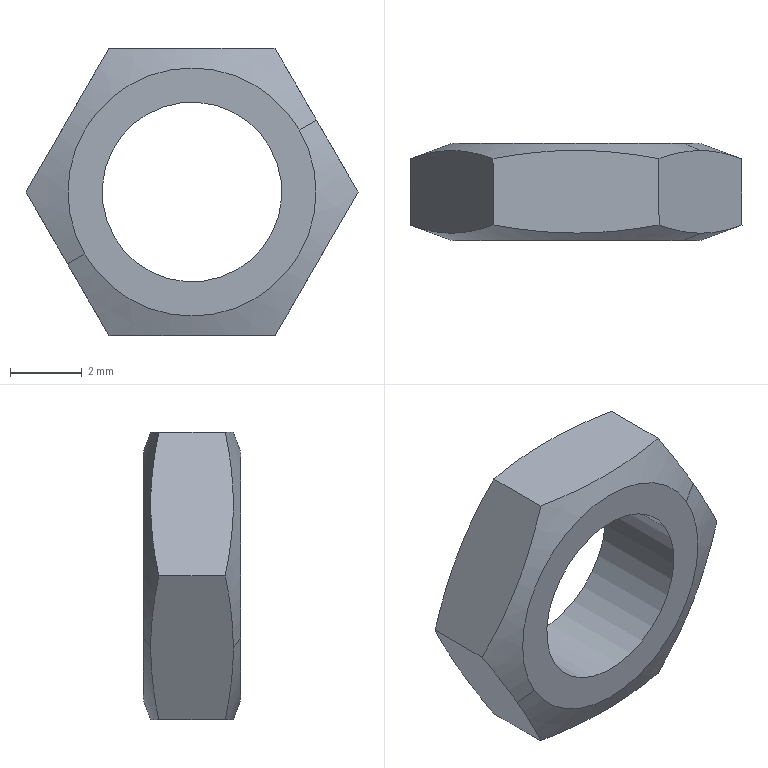Component | SolidWorks | 18M5StainlessSteelNut-1 | 1 solid | 14 faces | box 9.24 x 2.7 x 8 mm | volume 91 mm3 | plane 8 | cone 4 | cylinder 2 | commonest cylinder face diameters 5 x2 | material SUS304
STEP:
#1=CARTESIAN_POINT('',(-0.6207,1.188,3.061));
#2=VERTEX_POINT('',#1);
#3=CARTESIAN_POINT('',(-0.4502,1.188,3.159));
#4=VERTEX_POINT('',#3);
#5=CARTESIAN_POINT('',(-0.5354,1.188,3.11));
#6=DIRECTION('',(0.,-1.,0.));
#7=DIRECTION('',(0.866,0.,0.5));
#8=AXIS2_PLACEMENT_3D('',#5,#6,#7);
#9=CIRCLE('',#8,0.09843);
#10=EDGE_CURVE('',#2,#4,#9,.T.);
#11=ORIENTED_EDGE('',*,*,#10,.F.);
#12=CARTESIAN_POINT('',(-0.6207,1.082,3.061));
#13=VERTEX_POINT('',#12);
#14=CARTESIAN_POINT('',(-0.6207,1.188,3.061));
#15=DIRECTION('',(0.,-1.,0.));
#16=VECTOR('',#15,39.37);
#17=LINE('',#14,#16);
#18=EDGE_CURVE('',#2,#13,#17,.T.);
#19=ORIENTED_EDGE('',*,*,#18,.T.);
#20=CARTESIAN_POINT('',(-0.4502,1.082,3.159));
#21=VERTEX_POINT('',#20);
#22=CARTESIAN_POINT('',(-0.5354,1.082,3.11));
#23=DIRECTION('',(0.,-1.,0.));
#24=DIRECTION('',(0.866,0.,0.5));
#25=AXIS2_PLACEMENT_3D('',#22,#23,#24);
#26=CIRCLE('',#25,0.09843);
#27=EDGE_CURVE('',#13,#21,#26,.T.);
#28=ORIENTED_EDGE('',*,*,#27,.T.);
#29=CARTESIAN_POINT('',(-0.4502,1.188,3.159));
#30=DIRECTION('',(0.,-1.,0.));
#31=VECTOR('',#30,39.37);
#32=LINE('',#29,#31);
#33=EDGE_CURVE('',#4,#21,#32,.T.);
#34=ORIENTED_EDGE('',*,*,#33,.F.);
#35=EDGE_LOOP('',(#11,#19,#28,#34));
#36=FACE_OUTER_BOUND('',#35,.T.);
#37=CARTESIAN_POINT('',(-0.5354,1.188,3.11));
#38=DIRECTION('',(0.,-1.,0.));
#39=DIRECTION('',(0.866,0.,0.5));
#40=AXIS2_PLACEMENT_3D('',#37,#38,#39);
#41=CYLINDRICAL_SURFACE('',#40,0.09843);
#42=ADVANCED_FACE('',(#36),#41,.F.);
#43=CARTESIAN_POINT('',(-0.4178,1.082,3.178));
#44=VERTEX_POINT('',#43);
#45=CARTESIAN_POINT('',(-0.653,1.082,3.042));
#46=VERTEX_POINT('',#45);
#47=CARTESIAN_POINT('',(-0.5354,1.082,3.11));
#48=DIRECTION('',(0.,-1.,0.));
#49=DIRECTION('',(-0.866,0.,-0.5));
#50=AXIS2_PLACEMENT_3D('',#47,#48,#49);
#51=CIRCLE('',#50,0.1358);
#52=EDGE_CURVE('',#44,#46,#51,.T.);
#53=ORIENTED_EDGE('',*,*,#52,.F.);
#54=CARTESIAN_POINT('',(-0.399,1.089,3.189));
#55=VERTEX_POINT('',#54);
#56=CARTESIAN_POINT('',(-0.3777,1.098,3.201));
#57=DIRECTION('',(0.8138,0.342,0.4698));
#58=VECTOR('',#57,39.37);
#59=LINE('',#56,#58);
#60=EDGE_CURVE('',#44,#55,#59,.T.);
#61=ORIENTED_EDGE('',*,*,#60,.T.);
#62=CARTESIAN_POINT('',(-0.4445,1.098,3.268));
#63=VERTEX_POINT('',#62);
#64=CARTESIAN_POINT('',(-0.399,1.089,3.189));
#65=CARTESIAN_POINT('',(-0.4142,1.089,3.215));
#66=CARTESIAN_POINT('',(-0.4293,1.093,3.241));
#67=CARTESIAN_POINT('',(-0.4445,1.098,3.268));
#68=B_SPLINE_CURVE_WITH_KNOTS('',3,(#64,#65,#66,#67),.UNSPECIFIED.,.F.,.F.,(4,4),(0.002309,0.004619),.UNSPECIFIED.);
#69=EDGE_CURVE('',#55,#63,#68,.T.);
#70=ORIENTED_EDGE('',*,*,#69,.T.);
#71=CARTESIAN_POINT('',(-0.6263,1.098,3.268));
#72=VERTEX_POINT('',#71);
#73=CARTESIAN_POINT('',(-0.4445,1.098,3.268));
#74=CARTESIAN_POINT('',(-0.4748,1.093,3.268));
#75=CARTESIAN_POINT('',(-0.5354,1.086,3.268));
#76=CARTESIAN_POINT('',(-0.596,1.093,3.268));
#77=CARTESIAN_POINT('',(-0.6263,1.098,3.268));
#78=B_SPLINE_CURVE_WITH_KNOTS('',3,(#73,#74,#75,#76,#77),.UNSPECIFIED.,.F.,.F.,(4,1,4),(0.,0.002309,0.004619),.UNSPECIFIED.);
#79=EDGE_CURVE('',#63,#72,#78,.T.);
#80=ORIENTED_EDGE('',*,*,#79,.T.);
#81=CARTESIAN_POINT('',(-0.7173,1.098,3.11));
#82=VERTEX_POINT('',#81);
#83=CARTESIAN_POINT('',(-0.6263,1.098,3.268));
#84=CARTESIAN_POINT('',(-0.6415,1.093,3.241));
#85=CARTESIAN_POINT('',(-0.6718,1.086,3.189));
#86=CARTESIAN_POINT('',(-0.7021,1.093,3.136));
#87=CARTESIAN_POINT('',(-0.7173,1.098,3.11));
#88=B_SPLINE_CURVE_WITH_KNOTS('',3,(#83,#84,#85,#86,#87),.UNSPECIFIED.,.F.,.F.,(4,1,4),(0.,0.002309,0.004619),.UNSPECIFIED.);
#89=EDGE_CURVE('',#72,#82,#88,.T.);
#90=ORIENTED_EDGE('',*,*,#89,.T.);
#91=CARTESIAN_POINT('',(-0.6718,1.089,3.031));
#92=VERTEX_POINT('',#91);
#93=CARTESIAN_POINT('',(-0.7173,1.098,3.11));
#94=CARTESIAN_POINT('',(-0.7021,1.093,3.084));
#95=CARTESIAN_POINT('',(-0.687,1.089,3.058));
#96=CARTESIAN_POINT('',(-0.6718,1.089,3.031));
#97=B_SPLINE_CURVE_WITH_KNOTS('',3,(#93,#94,#95,#96),.UNSPECIFIED.,.F.,.F.,(4,4),(0.,0.002309),.UNSPECIFIED.);
#98=EDGE_CURVE('',#82,#92,#97,.T.);
#99=ORIENTED_EDGE('',*,*,#98,.T.);
#100=CARTESIAN_POINT('',(-0.6931,1.098,3.019));
#101=DIRECTION('',(-0.8138,0.342,-0.4698));
#102=VECTOR('',#101,39.37);
#103=LINE('',#100,#102);
#104=EDGE_CURVE('',#46,#92,#103,.T.);
#105=ORIENTED_EDGE('',*,*,#104,.F.);
#106=EDGE_LOOP('',(#53,#61,#70,#80,#90,#99,#105));
#107=FACE_OUTER_BOUND('',#106,.T.);
#108=CARTESIAN_POINT('',(-0.5354,1.098,3.11));
#109=DIRECTION('',(-0.,1.,-0.));
#110=DIRECTION('',(-0.866,0.,-0.5));
#111=AXIS2_PLACEMENT_3D('',#108,#109,#110);
#112=CONICAL_SURFACE('',#111,0.1821,1.222);
#113=ADVANCED_FACE('',(#107),#112,.T.);
#114=CARTESIAN_POINT('',(-0.4178,1.188,3.178));
#115=VERTEX_POINT('',#114);
#116=CARTESIAN_POINT('',(-0.653,1.188,3.042));
#117=VERTEX_POINT('',#116);
#118=CARTESIAN_POINT('',(-0.5354,1.188,3.11));
#119=DIRECTION('',(0.,-1.,0.));
#120=DIRECTION('',(0.866,0.,0.5));
#121=AXIS2_PLACEMENT_3D('',#118,#119,#120);
#122=CIRCLE('',#121,0.1358);
#123=EDGE_CURVE('',#115,#117,#122,.T.);
#124=ORIENTED_EDGE('',*,*,#123,.T.);
#125=CARTESIAN_POINT('',(-0.6718,1.18,3.031));
#126=VERTEX_POINT('',#125);
#127=CARTESIAN_POINT('',(-0.6931,1.171,3.019));
#128=DIRECTION('',(-0.8138,-0.342,-0.4698));
#129=VECTOR('',#128,39.37);
#130=LINE('',#127,#129);
#131=EDGE_CURVE('',#117,#126,#130,.T.);
#132=ORIENTED_EDGE('',*,*,#131,.T.);
#133=CARTESIAN_POINT('',(-0.7173,1.171,3.11));
#134=VERTEX_POINT('',#133);
#135=CARTESIAN_POINT('',(-0.6718,1.18,3.031));
#136=CARTESIAN_POINT('',(-0.687,1.18,3.058));
#137=CARTESIAN_POINT('',(-0.7021,1.177,3.084));
#138=CARTESIAN_POINT('',(-0.7173,1.171,3.11));
#139=B_SPLINE_CURVE_WITH_KNOTS('',3,(#135,#136,#137,#138),.UNSPECIFIED.,.F.,.F.,(4,4),(0.002309,0.004619),.UNSPECIFIED.);
#140=EDGE_CURVE('',#126,#134,#139,.T.);
#141=ORIENTED_EDGE('',*,*,#140,.T.);
#142=CARTESIAN_POINT('',(-0.6263,1.171,3.268));
#143=VERTEX_POINT('',#142);
#144=CARTESIAN_POINT('',(-0.7173,1.171,3.11));
#145=CARTESIAN_POINT('',(-0.7021,1.177,3.136));
#146=CARTESIAN_POINT('',(-0.6718,1.183,3.189));
#147=CARTESIAN_POINT('',(-0.6415,1.177,3.241));
#148=CARTESIAN_POINT('',(-0.6263,1.171,3.268));
#149=B_SPLINE_CURVE_WITH_KNOTS('',3,(#144,#145,#146,#147,#148),.UNSPECIFIED.,.F.,.F.,(4,1,4),(0.,0.002309,0.004619),.UNSPECIFIED.);
#150=EDGE_CURVE('',#134,#143,#149,.T.);
#151=ORIENTED_EDGE('',*,*,#150,.T.);
#152=CARTESIAN_POINT('',(-0.4445,1.171,3.268));
#153=VERTEX_POINT('',#152);
#154=CARTESIAN_POINT('',(-0.6263,1.171,3.268));
#155=CARTESIAN_POINT('',(-0.596,1.177,3.268));
#156=CARTESIAN_POINT('',(-0.5354,1.183,3.268));
#157=CARTESIAN_POINT('',(-0.4748,1.177,3.268));
#158=CARTESIAN_POINT('',(-0.4445,1.171,3.268));
#159=B_SPLINE_CURVE_WITH_KNOTS('',3,(#154,#155,#156,#157,#158),.UNSPECIFIED.,.F.,.F.,(4,1,4),(0.,0.002309,0.004619),.UNSPECIFIED.);
#160=EDGE_CURVE('',#143,#153,#159,.T.);
#161=ORIENTED_EDGE('',*,*,#160,.T.);
#162=CARTESIAN_POINT('',(-0.399,1.18,3.189));
#163=VERTEX_POINT('',#162);
#164=CARTESIAN_POINT('',(-0.4445,1.171,3.268));
#165=CARTESIAN_POINT('',(-0.4293,1.177,3.241));
#166=CARTESIAN_POINT('',(-0.4142,1.18,3.215));
#167=CARTESIAN_POINT('',(-0.399,1.18,3.189));
#168=B_SPLINE_CURVE_WITH_KNOTS('',3,(#164,#165,#166,#167),.UNSPECIFIED.,.F.,.F.,(4,4),(0.,0.002309),.UNSPECIFIED.);
#169=EDGE_CURVE('',#153,#163,#168,.T.);
#170=ORIENTED_EDGE('',*,*,#169,.T.);
#171=CARTESIAN_POINT('',(-0.3777,1.171,3.201));
#172=DIRECTION('',(0.8138,-0.342,0.4698));
#173=VECTOR('',#172,39.37);
#174=LINE('',#171,#173);
#175=EDGE_CURVE('',#115,#163,#174,.T.);
#176=ORIENTED_EDGE('',*,*,#175,.F.);
#177=EDGE_LOOP('',(#124,#132,#141,#151,#161,#170,#176));
#178=FACE_OUTER_BOUND('',#177,.T.);
#179=CARTESIAN_POINT('',(-0.5354,1.171,3.11));
#180=DIRECTION('',(0.,-1.,0.));
#181=DIRECTION('',(0.866,0.,0.5));
#182=AXIS2_PLACEMENT_3D('',#179,#180,#181);
#183=CONICAL_SURFACE('',#182,0.1821,1.222);
#184=ADVANCED_FACE('',(#178),#183,.T.);
#185=ORIENTED_EDGE('',*,*,#123,.F.);
#186=CARTESIAN_POINT('',(-0.5354,1.188,3.11));
#187=DIRECTION('',(0.,-1.,0.));
#188=DIRECTION('',(0.866,0.,0.5));
#189=AXIS2_PLACEMENT_3D('',#186,#187,#188);
#190=CIRCLE('',#189,0.1358);
#191=EDGE_CURVE('',#117,#115,#190,.T.);
#192=ORIENTED_EDGE('',*,*,#191,.F.);
#193=EDGE_LOOP('',(#185,#192));
#194=FACE_OUTER_BOUND('',#193,.T.);
#195=CARTESIAN_POINT('',(-0.5354,1.188,3.11));
#196=DIRECTION('',(0.,-1.,0.));
#197=DIRECTION('',(0.866,0.,0.5));
#198=AXIS2_PLACEMENT_3D('',#195,#196,#197);
#199=CIRCLE('',#198,0.09843);
#200=EDGE_CURVE('',#4,#2,#199,.T.);
#201=ORIENTED_EDGE('',*,*,#200,.T.);
#202=ORIENTED_EDGE('',*,*,#10,.T.);
#203=EDGE_LOOP('',(#201,#202));
#204=FACE_BOUND('',#203,.T.);
#205=CARTESIAN_POINT('',(-0.5354,1.188,3.11));
#206=DIRECTION('',(0.,-1.,0.));
#207=DIRECTION('',(0.866,0.,0.5));
#208=AXIS2_PLACEMENT_3D('',#205,#206,#207);
#209=PLANE('',#208);
#210=ADVANCED_FACE('',(#194,#204),#209,.F.);
#211=CARTESIAN_POINT('',(-0.5354,1.082,3.11));
#212=DIRECTION('',(0.,-1.,0.));
#213=DIRECTION('',(0.866,0.,0.5));
#214=AXIS2_PLACEMENT_3D('',#211,#212,#213);
#215=CIRCLE('',#214,0.09843);
#216=EDGE_CURVE('',#21,#13,#215,.T.);
#217=ORIENTED_EDGE('',*,*,#216,.F.);
#218=ORIENTED_EDGE('',*,*,#27,.F.);
#219=EDGE_LOOP('',(#217,#218));
#220=FACE_BOUND('',#219,.T.);
#221=CARTESIAN_POINT('',(-0.5354,1.082,3.11));
#222=DIRECTION('',(0.,-1.,0.));
#223=DIRECTION('',(-0.866,0.,-0.5));
#224=AXIS2_PLACEMENT_3D('',#221,#222,#223);
#225=CIRCLE('',#224,0.1358);
#226=EDGE_CURVE('',#46,#44,#225,.T.);
#227=ORIENTED_EDGE('',*,*,#226,.T.);
#228=ORIENTED_EDGE('',*,*,#52,.T.);
#229=EDGE_LOOP('',(#227,#228));
#230=FACE_OUTER_BOUND('',#229,.T.);
#231=CARTESIAN_POINT('',(-0.5354,1.082,3.11));
#232=DIRECTION('',(0.,-1.,0.));
#233=DIRECTION('',(0.866,0.,0.5));
#234=AXIS2_PLACEMENT_3D('',#231,#232,#233);
#235=PLANE('',#234);
#236=ADVANCED_FACE('',(#220,#230),#235,.T.);
#237=ORIENTED_EDGE('',*,*,#60,.F.);
#238=ORIENTED_EDGE('',*,*,#226,.F.);
#239=ORIENTED_EDGE('',*,*,#104,.T.);
#240=CARTESIAN_POINT('',(-0.6263,1.098,2.953));
#241=VERTEX_POINT('',#240);
#242=CARTESIAN_POINT('',(-0.6718,1.089,3.031));
#243=CARTESIAN_POINT('',(-0.6566,1.089,3.005));
#244=CARTESIAN_POINT('',(-0.6415,1.093,2.979));
#245=CARTESIAN_POINT('',(-0.6263,1.098,2.953));
#246=B_SPLINE_CURVE_WITH_KNOTS('',3,(#242,#243,#244,#245),.UNSPECIFIED.,.F.,.F.,(4,4),(0.002309,0.004619),.UNSPECIFIED.);
#247=EDGE_CURVE('',#92,#241,#246,.T.);
#248=ORIENTED_EDGE('',*,*,#247,.T.);
#249=CARTESIAN_POINT('',(-0.4445,1.098,2.953));
#250=VERTEX_POINT('',#249);
#251=CARTESIAN_POINT('',(-0.6263,1.098,2.953));
#252=CARTESIAN_POINT('',(-0.596,1.093,2.953));
#253=CARTESIAN_POINT('',(-0.5354,1.086,2.953));
#254=CARTESIAN_POINT('',(-0.4748,1.093,2.953));
#255=CARTESIAN_POINT('',(-0.4445,1.098,2.953));
#256=B_SPLINE_CURVE_WITH_KNOTS('',3,(#251,#252,#253,#254,#255),.UNSPECIFIED.,.F.,.F.,(4,1,4),(0.,0.002309,0.004619),.UNSPECIFIED.);
#257=EDGE_CURVE('',#241,#250,#256,.T.);
#258=ORIENTED_EDGE('',*,*,#257,.T.);
#259=CARTESIAN_POINT('',(-0.3536,1.098,3.11));
#260=VERTEX_POINT('',#259);
#261=CARTESIAN_POINT('',(-0.4445,1.098,2.953));
#262=CARTESIAN_POINT('',(-0.4293,1.093,2.979));
#263=CARTESIAN_POINT('',(-0.399,1.086,3.031));
#264=CARTESIAN_POINT('',(-0.3687,1.093,3.084));
#265=CARTESIAN_POINT('',(-0.3536,1.098,3.11));
#266=B_SPLINE_CURVE_WITH_KNOTS('',3,(#261,#262,#263,#264,#265),.UNSPECIFIED.,.F.,.F.,(4,1,4),(0.,0.002309,0.004619),.UNSPECIFIED.);
#267=EDGE_CURVE('',#250,#260,#266,.T.);
#268=ORIENTED_EDGE('',*,*,#267,.T.);
#269=CARTESIAN_POINT('',(-0.3536,1.098,3.11));
#270=CARTESIAN_POINT('',(-0.3687,1.093,3.136));
#271=CARTESIAN_POINT('',(-0.3839,1.089,3.163));
#272=CARTESIAN_POINT('',(-0.399,1.089,3.189));
#273=B_SPLINE_CURVE_WITH_KNOTS('',3,(#269,#270,#271,#272),.UNSPECIFIED.,.F.,.F.,(4,4),(0.,0.002309),.UNSPECIFIED.);
#274=EDGE_CURVE('',#260,#55,#273,.T.);
#275=ORIENTED_EDGE('',*,*,#274,.T.);
#276=EDGE_LOOP('',(#237,#238,#239,#248,#258,#268,#275));
#277=FACE_OUTER_BOUND('',#276,.T.);
#278=CARTESIAN_POINT('',(-0.5354,1.098,3.11));
#279=DIRECTION('',(-0.,1.,-0.));
#280=DIRECTION('',(-0.866,0.,-0.5));
#281=AXIS2_PLACEMENT_3D('',#278,#279,#280);
#282=CONICAL_SURFACE('',#281,0.1821,1.222);
#283=ADVANCED_FACE('',(#277),#282,.T.);
#284=ORIENTED_EDGE('',*,*,#131,.F.);
#285=ORIENTED_EDGE('',*,*,#191,.T.);
#286=ORIENTED_EDGE('',*,*,#175,.T.);
#287=CARTESIAN_POINT('',(-0.3536,1.171,3.11));
#288=VERTEX_POINT('',#287);
#289=CARTESIAN_POINT('',(-0.399,1.18,3.189));
#290=CARTESIAN_POINT('',(-0.3839,1.18,3.163));
#291=CARTESIAN_POINT('',(-0.3687,1.177,3.136));
#292=CARTESIAN_POINT('',(-0.3536,1.171,3.11));
#293=B_SPLINE_CURVE_WITH_KNOTS('',3,(#289,#290,#291,#292),.UNSPECIFIED.,.F.,.F.,(4,4),(0.002309,0.004619),.UNSPECIFIED.);
#294=EDGE_CURVE('',#163,#288,#293,.T.);
#295=ORIENTED_EDGE('',*,*,#294,.T.);
#296=CARTESIAN_POINT('',(-0.4445,1.171,2.953));
#297=VERTEX_POINT('',#296);
#298=CARTESIAN_POINT('',(-0.3536,1.171,3.11));
#299=CARTESIAN_POINT('',(-0.3687,1.177,3.084));
#300=CARTESIAN_POINT('',(-0.399,1.183,3.031));
#301=CARTESIAN_POINT('',(-0.4293,1.177,2.979));
#302=CARTESIAN_POINT('',(-0.4445,1.171,2.953));
#303=B_SPLINE_CURVE_WITH_KNOTS('',3,(#298,#299,#300,#301,#302),.UNSPECIFIED.,.F.,.F.,(4,1,4),(0.,0.002309,0.004619),.UNSPECIFIED.);
#304=EDGE_CURVE('',#288,#297,#303,.T.);
#305=ORIENTED_EDGE('',*,*,#304,.T.);
#306=CARTESIAN_POINT('',(-0.6263,1.171,2.953));
#307=VERTEX_POINT('',#306);
#308=CARTESIAN_POINT('',(-0.4445,1.171,2.953));
#309=CARTESIAN_POINT('',(-0.4748,1.177,2.953));
#310=CARTESIAN_POINT('',(-0.5354,1.183,2.953));
#311=CARTESIAN_POINT('',(-0.596,1.177,2.953));
#312=CARTESIAN_POINT('',(-0.6263,1.171,2.953));
#313=B_SPLINE_CURVE_WITH_KNOTS('',3,(#308,#309,#310,#311,#312),.UNSPECIFIED.,.F.,.F.,(4,1,4),(0.,0.002309,0.004619),.UNSPECIFIED.);
#314=EDGE_CURVE('',#297,#307,#313,.T.);
#315=ORIENTED_EDGE('',*,*,#314,.T.);
#316=CARTESIAN_POINT('',(-0.6263,1.171,2.953));
#317=CARTESIAN_POINT('',(-0.6415,1.177,2.979));
#318=CARTESIAN_POINT('',(-0.6566,1.18,3.005));
#319=CARTESIAN_POINT('',(-0.6718,1.18,3.031));
#320=B_SPLINE_CURVE_WITH_KNOTS('',3,(#316,#317,#318,#319),.UNSPECIFIED.,.F.,.F.,(4,4),(0.,0.002309),.UNSPECIFIED.);
#321=EDGE_CURVE('',#307,#126,#320,.T.);
#322=ORIENTED_EDGE('',*,*,#321,.T.);
#323=EDGE_LOOP('',(#284,#285,#286,#295,#305,#315,#322));
#324=FACE_OUTER_BOUND('',#323,.T.);
#325=CARTESIAN_POINT('',(-0.5354,1.171,3.11));
#326=DIRECTION('',(0.,-1.,0.));
#327=DIRECTION('',(0.866,0.,0.5));
#328=AXIS2_PLACEMENT_3D('',#325,#326,#327);
#329=CONICAL_SURFACE('',#328,0.1821,1.222);
#330=ADVANCED_FACE('',(#324),#329,.T.);
#331=ORIENTED_EDGE('',*,*,#274,.F.);
#332=CARTESIAN_POINT('',(-0.3536,1.082,3.11));
#333=DIRECTION('',(0.,-1.,0.));
#334=VECTOR('',#333,39.37);
#335=LINE('',#332,#334);
#336=EDGE_CURVE('',#288,#260,#335,.T.);
#337=ORIENTED_EDGE('',*,*,#336,.F.);
#338=ORIENTED_EDGE('',*,*,#294,.F.);
#339=ORIENTED_EDGE('',*,*,#169,.F.);
#340=CARTESIAN_POINT('',(-0.4445,1.082,3.268));
#341=DIRECTION('',(-0.,1.,-0.));
#342=VECTOR('',#341,39.37);
#343=LINE('',#340,#342);
#344=EDGE_CURVE('',#63,#153,#343,.T.);
#345=ORIENTED_EDGE('',*,*,#344,.F.);
#346=ORIENTED_EDGE('',*,*,#69,.F.);
#347=EDGE_LOOP('',(#331,#337,#338,#339,#345,#346));
#348=FACE_OUTER_BOUND('',#347,.T.);
#349=CARTESIAN_POINT('',(-0.3536,1.082,3.11));
#350=DIRECTION('',(-0.866,-0.,-0.5));
#351=DIRECTION('',(0.,-1.,0.));
#352=AXIS2_PLACEMENT_3D('',#349,#350,#351);
#353=PLANE('',#352);
#354=ADVANCED_FACE('',(#348),#353,.F.);
#355=ORIENTED_EDGE('',*,*,#267,.F.);
#356=CARTESIAN_POINT('',(-0.4445,1.082,2.953));
#357=DIRECTION('',(0.,-1.,0.));
#358=VECTOR('',#357,39.37);
#359=LINE('',#356,#358);
#360=EDGE_CURVE('',#297,#250,#359,.T.);
#361=ORIENTED_EDGE('',*,*,#360,.F.);
#362=ORIENTED_EDGE('',*,*,#304,.F.);
#363=ORIENTED_EDGE('',*,*,#336,.T.);
#364=EDGE_LOOP('',(#355,#361,#362,#363));
#365=FACE_OUTER_BOUND('',#364,.T.);
#366=CARTESIAN_POINT('',(-0.4445,1.082,2.953));
#367=DIRECTION('',(-0.866,-0.,0.5));
#368=DIRECTION('',(-0.5,-0.,-0.866));
#369=AXIS2_PLACEMENT_3D('',#366,#367,#368);
#370=PLANE('',#369);
#371=ADVANCED_FACE('',(#365),#370,.F.);
#372=ORIENTED_EDGE('',*,*,#257,.F.);
#373=CARTESIAN_POINT('',(-0.6263,1.082,2.953));
#374=DIRECTION('',(0.,-1.,0.));
#375=VECTOR('',#374,39.37);
#376=LINE('',#373,#375);
#377=EDGE_CURVE('',#307,#241,#376,.T.);
#378=ORIENTED_EDGE('',*,*,#377,.F.);
#379=ORIENTED_EDGE('',*,*,#314,.F.);
#380=ORIENTED_EDGE('',*,*,#360,.T.);
#381=EDGE_LOOP('',(#372,#378,#379,#380));
#382=FACE_OUTER_BOUND('',#381,.T.);
#383=CARTESIAN_POINT('',(-0.6263,1.082,2.953));
#384=DIRECTION('',(-0.,0.,1.));
#385=DIRECTION('',(-1.,-0.,0.));
#386=AXIS2_PLACEMENT_3D('',#383,#384,#385);
#387=PLANE('',#386);
#388=ADVANCED_FACE('',(#382),#387,.F.);
#389=ORIENTED_EDGE('',*,*,#98,.F.);
#390=CARTESIAN_POINT('',(-0.7173,1.082,3.11));
#391=DIRECTION('',(0.,-1.,0.));
#392=VECTOR('',#391,39.37);
#393=LINE('',#390,#392);
#394=EDGE_CURVE('',#134,#82,#393,.T.);
#395=ORIENTED_EDGE('',*,*,#394,.F.);
#396=ORIENTED_EDGE('',*,*,#140,.F.);
#397=ORIENTED_EDGE('',*,*,#321,.F.);
#398=ORIENTED_EDGE('',*,*,#377,.T.);
#399=ORIENTED_EDGE('',*,*,#247,.F.);
#400=EDGE_LOOP('',(#389,#395,#396,#397,#398,#399));
#401=FACE_OUTER_BOUND('',#400,.T.);
#402=CARTESIAN_POINT('',(-0.7173,1.082,3.11));
#403=DIRECTION('',(0.866,0.,0.5));
#404=DIRECTION('',(-0.,1.,-0.));
#405=AXIS2_PLACEMENT_3D('',#402,#403,#404);
#406=PLANE('',#405);
#407=ADVANCED_FACE('',(#401),#406,.F.);
#408=ORIENTED_EDGE('',*,*,#89,.F.);
#409=CARTESIAN_POINT('',(-0.6263,1.082,3.268));
#410=DIRECTION('',(0.,-1.,0.));
#411=VECTOR('',#410,39.37);
#412=LINE('',#409,#411);
#413=EDGE_CURVE('',#143,#72,#412,.T.);
#414=ORIENTED_EDGE('',*,*,#413,.F.);
#415=ORIENTED_EDGE('',*,*,#150,.F.);
#416=ORIENTED_EDGE('',*,*,#394,.T.);
#417=EDGE_LOOP('',(#408,#414,#415,#416));
#418=FACE_OUTER_BOUND('',#417,.T.);
#419=CARTESIAN_POINT('',(-0.6263,1.082,3.268));
#420=DIRECTION('',(0.866,0.,-0.5));
#421=DIRECTION('',(0.5,0.,0.866));
#422=AXIS2_PLACEMENT_3D('',#419,#420,#421);
#423=PLANE('',#422);
#424=ADVANCED_FACE('',(#418),#423,.F.);
#425=ORIENTED_EDGE('',*,*,#79,.F.);
#426=ORIENTED_EDGE('',*,*,#344,.T.);
#427=ORIENTED_EDGE('',*,*,#160,.F.);
#428=ORIENTED_EDGE('',*,*,#413,.T.);
#429=EDGE_LOOP('',(#425,#426,#427,#428));
#430=FACE_OUTER_BOUND('',#429,.T.);
#431=CARTESIAN_POINT('',(-0.4445,1.082,3.268));
#432=DIRECTION('',(0.,-0.,-1.));
#433=DIRECTION('',(1.,0.,0.));
#434=AXIS2_PLACEMENT_3D('',#431,#432,#433);
#435=PLANE('',#434);
#436=ADVANCED_FACE('',(#430),#435,.F.);
#437=ORIENTED_EDGE('',*,*,#18,.F.);
#438=ORIENTED_EDGE('',*,*,#200,.F.);
#439=ORIENTED_EDGE('',*,*,#33,.T.);
#440=ORIENTED_EDGE('',*,*,#216,.T.);
#441=EDGE_LOOP('',(#437,#438,#439,#440));
#442=FACE_OUTER_BOUND('',#441,.T.);
#443=CARTESIAN_POINT('',(-0.5354,1.188,3.11));
#444=DIRECTION('',(0.,-1.,0.));
#445=DIRECTION('',(0.866,0.,0.5));
#446=AXIS2_PLACEMENT_3D('',#443,#444,#445);
#447=CYLINDRICAL_SURFACE('',#446,0.09843);
#448=ADVANCED_FACE('',(#442),#447,.F.);
#449=CLOSED_SHELL('',(#42,#113,#184,#210,#236,#283,#330,#354,#371,#388,#407,#424,#436,#448));
#450=MANIFOLD_SOLID_BREP('',#449);
#451=CARTESIAN_POINT('',(0.,0.,0.));
#452=DIRECTION('',(0.,0.,1.));
#453=DIRECTION('',(1.,0.,0.));
#454=AXIS2_PLACEMENT_3D('',#451,#452,#453);
#455=(LENGTH_UNIT()NAMED_UNIT(*)SI_UNIT($,.METRE.));
#456=LENGTH_MEASURE_WITH_UNIT(LENGTH_MEASURE(0.0254),#455);
#457=DIMENSIONAL_EXPONENTS(1.,0.,0.,0.,0.,0.,0.);
#458=(CONVERSION_BASED_UNIT('',#456)LENGTH_UNIT()NAMED_UNIT(#457));
#459=UNCERTAINTY_MEASURE_WITH_UNIT(LENGTH_MEASURE(0.00001),#458,'','');
#460=(NAMED_UNIT(*)PLANE_ANGLE_UNIT()SI_UNIT($,.RADIAN.));
#461=(NAMED_UNIT(*)SI_UNIT($,.STERADIAN.)SOLID_ANGLE_UNIT());
#462=(GEOMETRIC_REPRESENTATION_CONTEXT(3)GLOBAL_UNCERTAINTY_ASSIGNED_CONTEXT((#459))GLOBAL_UNIT_ASSIGNED_CONTEXT((#458,#460,#461))REPRESENTATION_CONTEXT('',''));
#463=ADVANCED_BREP_SHAPE_REPRESENTATION('',(#450,#454),#462);
#464=COLOUR_RGB('',0.7922,0.8196,0.9333);
#465=FILL_AREA_STYLE_COLOUR('',#464);
#466=FILL_AREA_STYLE('',(#465));
#467=SURFACE_STYLE_FILL_AREA(#466);
#468=SURFACE_SIDE_STYLE('',(#467));
#469=SURFACE_STYLE_USAGE(.BOTH.,#468);
#470=PRESENTATION_STYLE_ASSIGNMENT((#469));
#471=STYLED_ITEM('',(#470),#450);
#472=(LENGTH_UNIT()NAMED_UNIT(*)SI_UNIT($,.METRE.));
#473=LENGTH_MEASURE_WITH_UNIT(LENGTH_MEASURE(0.0254),#472);
#474=DIMENSIONAL_EXPONENTS(1.,0.,0.,0.,0.,0.,0.);
#475=(CONVERSION_BASED_UNIT('',#473)LENGTH_UNIT()NAMED_UNIT(#474));
#476=UNCERTAINTY_MEASURE_WITH_UNIT(LENGTH_MEASURE(0.00001),#475,'','');
#477=(NAMED_UNIT(*)PLANE_ANGLE_UNIT()SI_UNIT($,.RADIAN.));
#478=(NAMED_UNIT(*)SI_UNIT($,.STERADIAN.)SOLID_ANGLE_UNIT());
#479=(GEOMETRIC_REPRESENTATION_CONTEXT(3)GLOBAL_UNCERTAINTY_ASSIGNED_CONTEXT((#476))GLOBAL_UNIT_ASSIGNED_CONTEXT((#475,#477,#478))REPRESENTATION_CONTEXT('',''));
#480=MECHANICAL_DESIGN_GEOMETRIC_PRESENTATION_REPRESENTATION('',(#471),#479);
#481=PRESENTATION_LAYER_ASSIGNMENT('','',(#471));